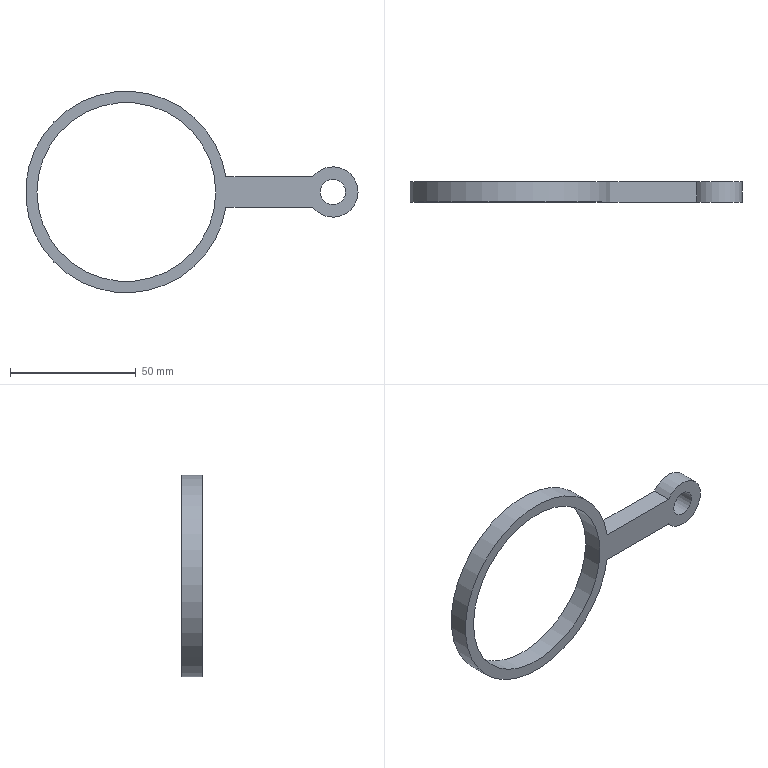Component | NX | ECCENTRIC_ROD | 1 solid | 8 faces | box 132 x 8 x 80 mm | volume 13571 mm3 | cylinder 4 | plane 4 | commonest cylinder face diameters 80 x1 20 x1 71 x1 10 x1
STEP:
#1=CARTESIAN_POINT('',(0.,0.,0.));
#2=DIRECTION('',(0.,0.,1.));
#3=DIRECTION('',(1.,0.,0.));
#4=AXIS2_PLACEMENT_3D('',#1,#2,#3);
#5=CARTESIAN_POINT('',(-111.854,-17.005,113.207));
#6=VERTEX_POINT('',#5);
#7=CARTESIAN_POINT('',(-111.854,-17.005,101.207));
#8=VERTEX_POINT('',#7);
#9=CARTESIAN_POINT('',(-151.401,-17.005,107.207));
#10=DIRECTION('',(0.,-1.,0.));
#11=DIRECTION('',(1.,0.,0.));
#12=AXIS2_PLACEMENT_3D('',#9,#10,#11);
#13=CIRCLE('',#12,40.);
#14=CARTESIAN_POINT('',(-151.401,-25.005,107.207));
#15=DIRECTION('',(0.,1.,0.));
#16=DIRECTION('',(-1.,0.,0.));
#17=AXIS2_PLACEMENT_3D('',#14,#15,#16);
#18=CYLINDRICAL_SURFACE('',#17,40.);
#19=CARTESIAN_POINT('',(3.142,8.));
#20=DIRECTION('',(-1.,0.));
#21=VECTOR('',#20,1.);
#22=LINE('',#19,#21);
#23=(GEOMETRIC_REPRESENTATION_CONTEXT(2)PARAMETRIC_REPRESENTATION_CONTEXT()REPRESENTATION_CONTEXT('',''));
#24=DEFINITIONAL_REPRESENTATION('',(#22),#23);
#25=PCURVE('',#18,#24);
#26=CARTESIAN_POINT('',(-151.401,-17.005,107.207));
#27=DIRECTION('',(0.,-1.,0.));
#28=DIRECTION('',(1.,0.,0.));
#29=AXIS2_PLACEMENT_3D('',#26,#27,#28);
#30=PLANE('',#29);
#31=CARTESIAN_POINT('',(0.,0.));
#32=DIRECTION('',(1.,0.));
#33=AXIS2_PLACEMENT_2D('',#31,#32);
#34=CIRCLE('',#33,40.);
#35=(GEOMETRIC_REPRESENTATION_CONTEXT(2)PARAMETRIC_REPRESENTATION_CONTEXT()REPRESENTATION_CONTEXT('',''));
#36=DEFINITIONAL_REPRESENTATION('',(#34),#35);
#37=PCURVE('',#30,#36);
#38=SURFACE_CURVE('',#13,(#25,#37),.PCURVE_S1.);
#39=EDGE_CURVE('',#6,#8,#38,.T.);
#40=ORIENTED_EDGE('',*,*,#39,.T.);
#41=CARTESIAN_POINT('',(-111.854,-25.005,101.207));
#42=VERTEX_POINT('',#41);
#43=CARTESIAN_POINT('',(-111.854,-25.005,101.207));
#44=DIRECTION('',(0.,1.,0.));
#45=VECTOR('',#44,1.);
#46=LINE('',#43,#45);
#47=CARTESIAN_POINT('',(-2.991,0.));
#48=DIRECTION('',(0.,1.));
#49=VECTOR('',#48,1.);
#50=LINE('',#47,#49);
#51=(GEOMETRIC_REPRESENTATION_CONTEXT(2)PARAMETRIC_REPRESENTATION_CONTEXT()REPRESENTATION_CONTEXT('',''));
#52=DEFINITIONAL_REPRESENTATION('',(#50),#51);
#53=PCURVE('',#18,#52);
#54=CARTESIAN_POINT('',(-111.854,-25.005,101.207));
#55=DIRECTION('',(-0.,0.,1.));
#56=DIRECTION('',(-1.,0.,-0.));
#57=AXIS2_PLACEMENT_3D('',#54,#55,#56);
#58=PLANE('',#57);
#59=CARTESIAN_POINT('',(0.,0.));
#60=DIRECTION('',(0.,-1.));
#61=VECTOR('',#60,1.);
#62=LINE('',#59,#61);
#63=(GEOMETRIC_REPRESENTATION_CONTEXT(2)PARAMETRIC_REPRESENTATION_CONTEXT()REPRESENTATION_CONTEXT('',''));
#64=DEFINITIONAL_REPRESENTATION('',(#62),#63);
#65=PCURVE('',#58,#64);
#66=SURFACE_CURVE('',#46,(#53,#65),.PCURVE_S1.);
#67=EDGE_CURVE('',#42,#8,#66,.T.);
#68=ORIENTED_EDGE('',*,*,#67,.F.);
#69=CARTESIAN_POINT('',(-111.854,-25.005,113.207));
#70=VERTEX_POINT('',#69);
#71=CARTESIAN_POINT('',(-151.401,-25.005,107.207));
#72=DIRECTION('',(0.,-1.,0.));
#73=DIRECTION('',(1.,0.,0.));
#74=AXIS2_PLACEMENT_3D('',#71,#72,#73);
#75=CIRCLE('',#74,40.);
#76=CARTESIAN_POINT('',(3.142,0.));
#77=DIRECTION('',(-1.,0.));
#78=VECTOR('',#77,1.);
#79=LINE('',#76,#78);
#80=(GEOMETRIC_REPRESENTATION_CONTEXT(2)PARAMETRIC_REPRESENTATION_CONTEXT()REPRESENTATION_CONTEXT('',''));
#81=DEFINITIONAL_REPRESENTATION('',(#79),#80);
#82=PCURVE('',#18,#81);
#83=CARTESIAN_POINT('',(-151.401,-25.005,107.207));
#84=DIRECTION('',(0.,-1.,0.));
#85=DIRECTION('',(1.,0.,0.));
#86=AXIS2_PLACEMENT_3D('',#83,#84,#85);
#87=PLANE('',#86);
#88=CARTESIAN_POINT('',(0.,0.));
#89=DIRECTION('',(1.,0.));
#90=AXIS2_PLACEMENT_2D('',#88,#89);
#91=CIRCLE('',#90,40.);
#92=(GEOMETRIC_REPRESENTATION_CONTEXT(2)PARAMETRIC_REPRESENTATION_CONTEXT()REPRESENTATION_CONTEXT('',''));
#93=DEFINITIONAL_REPRESENTATION('',(#91),#92);
#94=PCURVE('',#87,#93);
#95=SURFACE_CURVE('',#75,(#82,#94),.PCURVE_S1.);
#96=EDGE_CURVE('',#70,#42,#95,.T.);
#97=ORIENTED_EDGE('',*,*,#96,.F.);
#98=CARTESIAN_POINT('',(-111.854,-25.005,113.207));
#99=DIRECTION('',(0.,1.,0.));
#100=VECTOR('',#99,1.);
#101=LINE('',#98,#100);
#102=CARTESIAN_POINT('',(2.991,0.));
#103=DIRECTION('',(0.,1.));
#104=VECTOR('',#103,1.);
#105=LINE('',#102,#104);
#106=(GEOMETRIC_REPRESENTATION_CONTEXT(2)PARAMETRIC_REPRESENTATION_CONTEXT()REPRESENTATION_CONTEXT('',''));
#107=DEFINITIONAL_REPRESENTATION('',(#105),#106);
#108=PCURVE('',#18,#107);
#109=CARTESIAN_POINT('',(-77.401,-25.005,113.207));
#110=DIRECTION('',(0.,0.,-1.));
#111=DIRECTION('',(0.,1.,0.));
#112=AXIS2_PLACEMENT_3D('',#109,#110,#111);
#113=PLANE('',#112);
#114=CARTESIAN_POINT('',(0.,-34.453));
#115=DIRECTION('',(1.,0.));
#116=VECTOR('',#115,1.);
#117=LINE('',#114,#116);
#118=(GEOMETRIC_REPRESENTATION_CONTEXT(2)PARAMETRIC_REPRESENTATION_CONTEXT()REPRESENTATION_CONTEXT('',''));
#119=DEFINITIONAL_REPRESENTATION('',(#117),#118);
#120=PCURVE('',#113,#119);
#121=SURFACE_CURVE('',#101,(#108,#120),.PCURVE_S1.);
#122=EDGE_CURVE('',#70,#6,#121,.T.);
#123=ORIENTED_EDGE('',*,*,#122,.T.);
#124=EDGE_LOOP('',(#40,#68,#97,#123));
#125=FACE_BOUND('',#124,.T.);
#126=ADVANCED_FACE('',(#125),#18,.T.);
#127=CARTESIAN_POINT('',(-77.401,-17.005,101.207));
#128=VERTEX_POINT('',#127);
#129=CARTESIAN_POINT('',(-111.854,-17.005,101.207));
#130=DIRECTION('',(1.,0.,0.));
#131=VECTOR('',#130,1.);
#132=LINE('',#129,#131);
#133=CARTESIAN_POINT('',(0.,-8.));
#134=DIRECTION('',(-1.,0.));
#135=VECTOR('',#134,1.);
#136=LINE('',#133,#135);
#137=(GEOMETRIC_REPRESENTATION_CONTEXT(2)PARAMETRIC_REPRESENTATION_CONTEXT()REPRESENTATION_CONTEXT('',''));
#138=DEFINITIONAL_REPRESENTATION('',(#136),#137);
#139=PCURVE('',#58,#138);
#140=CARTESIAN_POINT('',(39.547,-6.));
#141=DIRECTION('',(1.,0.));
#142=VECTOR('',#141,1.);
#143=LINE('',#140,#142);
#144=(GEOMETRIC_REPRESENTATION_CONTEXT(2)PARAMETRIC_REPRESENTATION_CONTEXT()REPRESENTATION_CONTEXT('',''));
#145=DEFINITIONAL_REPRESENTATION('',(#143),#144);
#146=PCURVE('',#30,#145);
#147=SURFACE_CURVE('',#132,(#139,#146),.PCURVE_S1.);
#148=EDGE_CURVE('',#8,#128,#147,.T.);
#149=ORIENTED_EDGE('',*,*,#148,.T.);
#150=CARTESIAN_POINT('',(-77.401,-25.005,101.207));
#151=VERTEX_POINT('',#150);
#152=CARTESIAN_POINT('',(-77.401,-25.005,101.207));
#153=DIRECTION('',(0.,1.,0.));
#154=VECTOR('',#153,1.);
#155=LINE('',#152,#154);
#156=CARTESIAN_POINT('',(-34.453,0.));
#157=DIRECTION('',(0.,-1.));
#158=VECTOR('',#157,1.);
#159=LINE('',#156,#158);
#160=(GEOMETRIC_REPRESENTATION_CONTEXT(2)PARAMETRIC_REPRESENTATION_CONTEXT()REPRESENTATION_CONTEXT('',''));
#161=DEFINITIONAL_REPRESENTATION('',(#159),#160);
#162=PCURVE('',#58,#161);
#163=CARTESIAN_POINT('',(-69.401,-25.005,107.207));
#164=DIRECTION('',(0.,1.,0.));
#165=DIRECTION('',(-1.,0.,0.));
#166=AXIS2_PLACEMENT_3D('',#163,#164,#165);
#167=CYLINDRICAL_SURFACE('',#166,10.);
#168=CARTESIAN_POINT('',(5.64,0.));
#169=DIRECTION('',(0.,1.));
#170=VECTOR('',#169,1.);
#171=LINE('',#168,#170);
#172=(GEOMETRIC_REPRESENTATION_CONTEXT(2)PARAMETRIC_REPRESENTATION_CONTEXT()REPRESENTATION_CONTEXT('',''));
#173=DEFINITIONAL_REPRESENTATION('',(#171),#172);
#174=PCURVE('',#167,#173);
#175=SURFACE_CURVE('',#155,(#162,#174),.PCURVE_S1.);
#176=EDGE_CURVE('',#151,#128,#175,.T.);
#177=ORIENTED_EDGE('',*,*,#176,.F.);
#178=CARTESIAN_POINT('',(-111.854,-25.005,101.207));
#179=DIRECTION('',(1.,0.,0.));
#180=VECTOR('',#179,1.);
#181=LINE('',#178,#180);
#182=CARTESIAN_POINT('',(0.,0.));
#183=DIRECTION('',(-1.,0.));
#184=VECTOR('',#183,1.);
#185=LINE('',#182,#184);
#186=(GEOMETRIC_REPRESENTATION_CONTEXT(2)PARAMETRIC_REPRESENTATION_CONTEXT()REPRESENTATION_CONTEXT('',''));
#187=DEFINITIONAL_REPRESENTATION('',(#185),#186);
#188=PCURVE('',#58,#187);
#189=CARTESIAN_POINT('',(39.547,-6.));
#190=DIRECTION('',(1.,0.));
#191=VECTOR('',#190,1.);
#192=LINE('',#189,#191);
#193=(GEOMETRIC_REPRESENTATION_CONTEXT(2)PARAMETRIC_REPRESENTATION_CONTEXT()REPRESENTATION_CONTEXT('',''));
#194=DEFINITIONAL_REPRESENTATION('',(#192),#193);
#195=PCURVE('',#87,#194);
#196=SURFACE_CURVE('',#181,(#188,#195),.PCURVE_S1.);
#197=EDGE_CURVE('',#42,#151,#196,.T.);
#198=ORIENTED_EDGE('',*,*,#197,.F.);
#199=ORIENTED_EDGE('',*,*,#67,.T.);
#200=EDGE_LOOP('',(#149,#177,#198,#199));
#201=FACE_BOUND('',#200,.T.);
#202=ADVANCED_FACE('',(#201),#58,.F.);
#203=CARTESIAN_POINT('',(-77.401,-17.005,113.207));
#204=VERTEX_POINT('',#203);
#205=CARTESIAN_POINT('',(-69.401,-17.005,107.207));
#206=DIRECTION('',(0.,-1.,0.));
#207=DIRECTION('',(1.,0.,0.));
#208=AXIS2_PLACEMENT_3D('',#205,#206,#207);
#209=CIRCLE('',#208,10.);
#210=CARTESIAN_POINT('',(9.425,8.));
#211=DIRECTION('',(-1.,0.));
#212=VECTOR('',#211,1.);
#213=LINE('',#210,#212);
#214=(GEOMETRIC_REPRESENTATION_CONTEXT(2)PARAMETRIC_REPRESENTATION_CONTEXT()REPRESENTATION_CONTEXT('',''));
#215=DEFINITIONAL_REPRESENTATION('',(#213),#214);
#216=PCURVE('',#167,#215);
#217=CARTESIAN_POINT('',(82.,0.));
#218=DIRECTION('',(1.,0.));
#219=AXIS2_PLACEMENT_2D('',#217,#218);
#220=CIRCLE('',#219,10.);
#221=(GEOMETRIC_REPRESENTATION_CONTEXT(2)PARAMETRIC_REPRESENTATION_CONTEXT()REPRESENTATION_CONTEXT('',''));
#222=DEFINITIONAL_REPRESENTATION('',(#220),#221);
#223=PCURVE('',#30,#222);
#224=SURFACE_CURVE('',#209,(#216,#223),.PCURVE_S1.);
#225=EDGE_CURVE('',#128,#204,#224,.T.);
#226=ORIENTED_EDGE('',*,*,#225,.T.);
#227=CARTESIAN_POINT('',(-77.401,-25.005,113.207));
#228=VERTEX_POINT('',#227);
#229=CARTESIAN_POINT('',(-77.401,-25.005,113.207));
#230=DIRECTION('',(0.,1.,0.));
#231=VECTOR('',#230,1.);
#232=LINE('',#229,#231);
#233=CARTESIAN_POINT('',(0.6435,0.));
#234=DIRECTION('',(0.,1.));
#235=VECTOR('',#234,1.);
#236=LINE('',#233,#235);
#237=(GEOMETRIC_REPRESENTATION_CONTEXT(2)PARAMETRIC_REPRESENTATION_CONTEXT()REPRESENTATION_CONTEXT('',''));
#238=DEFINITIONAL_REPRESENTATION('',(#236),#237);
#239=PCURVE('',#167,#238);
#240=CARTESIAN_POINT('',(0.,0.));
#241=DIRECTION('',(1.,0.));
#242=VECTOR('',#241,1.);
#243=LINE('',#240,#242);
#244=(GEOMETRIC_REPRESENTATION_CONTEXT(2)PARAMETRIC_REPRESENTATION_CONTEXT()REPRESENTATION_CONTEXT('',''));
#245=DEFINITIONAL_REPRESENTATION('',(#243),#244);
#246=PCURVE('',#113,#245);
#247=SURFACE_CURVE('',#232,(#239,#246),.PCURVE_S1.);
#248=EDGE_CURVE('',#228,#204,#247,.T.);
#249=ORIENTED_EDGE('',*,*,#248,.F.);
#250=CARTESIAN_POINT('',(-69.401,-25.005,107.207));
#251=DIRECTION('',(0.,-1.,0.));
#252=DIRECTION('',(1.,0.,0.));
#253=AXIS2_PLACEMENT_3D('',#250,#251,#252);
#254=CIRCLE('',#253,10.);
#255=CARTESIAN_POINT('',(9.425,0.));
#256=DIRECTION('',(-1.,0.));
#257=VECTOR('',#256,1.);
#258=LINE('',#255,#257);
#259=(GEOMETRIC_REPRESENTATION_CONTEXT(2)PARAMETRIC_REPRESENTATION_CONTEXT()REPRESENTATION_CONTEXT('',''));
#260=DEFINITIONAL_REPRESENTATION('',(#258),#259);
#261=PCURVE('',#167,#260);
#262=CARTESIAN_POINT('',(82.,0.));
#263=DIRECTION('',(1.,0.));
#264=AXIS2_PLACEMENT_2D('',#262,#263);
#265=CIRCLE('',#264,10.);
#266=(GEOMETRIC_REPRESENTATION_CONTEXT(2)PARAMETRIC_REPRESENTATION_CONTEXT()REPRESENTATION_CONTEXT('',''));
#267=DEFINITIONAL_REPRESENTATION('',(#265),#266);
#268=PCURVE('',#87,#267);
#269=SURFACE_CURVE('',#254,(#261,#268),.PCURVE_S1.);
#270=EDGE_CURVE('',#151,#228,#269,.T.);
#271=ORIENTED_EDGE('',*,*,#270,.F.);
#272=ORIENTED_EDGE('',*,*,#176,.T.);
#273=EDGE_LOOP('',(#226,#249,#271,#272));
#274=FACE_BOUND('',#273,.T.);
#275=ADVANCED_FACE('',(#274),#167,.T.);
#276=CARTESIAN_POINT('',(-115.901,-25.005,107.207));
#277=VERTEX_POINT('',#276);
#278=CARTESIAN_POINT('',(-151.401,-25.005,107.207));
#279=DIRECTION('',(0.,-1.,0.));
#280=DIRECTION('',(1.,0.,0.));
#281=AXIS2_PLACEMENT_3D('',#278,#279,#280);
#282=CIRCLE('',#281,35.5);
#283=CARTESIAN_POINT('',(-151.401,-25.005,107.207));
#284=DIRECTION('',(0.,1.,0.));
#285=DIRECTION('',(-1.,0.,0.));
#286=AXIS2_PLACEMENT_3D('',#283,#284,#285);
#287=CYLINDRICAL_SURFACE('',#286,35.5);
#288=CARTESIAN_POINT('',(9.425,0.));
#289=DIRECTION('',(-1.,0.));
#290=VECTOR('',#289,1.);
#291=LINE('',#288,#290);
#292=(GEOMETRIC_REPRESENTATION_CONTEXT(2)PARAMETRIC_REPRESENTATION_CONTEXT()REPRESENTATION_CONTEXT('',''));
#293=DEFINITIONAL_REPRESENTATION('',(#291),#292);
#294=PCURVE('',#287,#293);
#295=CARTESIAN_POINT('',(0.,0.));
#296=DIRECTION('',(1.,0.));
#297=AXIS2_PLACEMENT_2D('',#295,#296);
#298=CIRCLE('',#297,35.5);
#299=(GEOMETRIC_REPRESENTATION_CONTEXT(2)PARAMETRIC_REPRESENTATION_CONTEXT()REPRESENTATION_CONTEXT('',''));
#300=DEFINITIONAL_REPRESENTATION('',(#298),#299);
#301=PCURVE('',#87,#300);
#302=SURFACE_CURVE('',#282,(#294,#301),.PCURVE_S1.);
#303=EDGE_CURVE('',#277,#277,#302,.T.);
#304=ORIENTED_EDGE('',*,*,#303,.F.);
#305=CARTESIAN_POINT('',(-115.901,-17.005,107.207));
#306=VERTEX_POINT('',#305);
#307=CARTESIAN_POINT('',(-115.901,-25.005,107.207));
#308=CARTESIAN_POINT('',(-115.901,-17.005,107.207));
#309=B_SPLINE_CURVE_WITH_KNOTS('',1,(#307,#308),.UNSPECIFIED.,.F.,.F.,(2,2),(0.,8.),.PIECEWISE_BEZIER_KNOTS.);
#310=CARTESIAN_POINT('',(9.425,0.));
#311=DIRECTION('',(0.,1.));
#312=VECTOR('',#311,1.);
#313=LINE('',#310,#312);
#314=(GEOMETRIC_REPRESENTATION_CONTEXT(2)PARAMETRIC_REPRESENTATION_CONTEXT()REPRESENTATION_CONTEXT('',''));
#315=DEFINITIONAL_REPRESENTATION('',(#313),#314);
#316=PCURVE('',#287,#315);
#317=CARTESIAN_POINT('',(3.142,0.));
#318=DIRECTION('',(0.,1.));
#319=VECTOR('',#318,1.);
#320=LINE('',#317,#319);
#321=(GEOMETRIC_REPRESENTATION_CONTEXT(2)PARAMETRIC_REPRESENTATION_CONTEXT()REPRESENTATION_CONTEXT('',''));
#322=DEFINITIONAL_REPRESENTATION('',(#320),#321);
#323=PCURVE('',#287,#322);
#324=SEAM_CURVE('',#309,(#316,#323),.PCURVE_S1.);
#325=EDGE_CURVE('',#277,#306,#324,.T.);
#326=ORIENTED_EDGE('',*,*,#325,.T.);
#327=CARTESIAN_POINT('',(-151.401,-17.005,107.207));
#328=DIRECTION('',(0.,-1.,0.));
#329=DIRECTION('',(1.,0.,0.));
#330=AXIS2_PLACEMENT_3D('',#327,#328,#329);
#331=CIRCLE('',#330,35.5);
#332=CARTESIAN_POINT('',(9.425,8.));
#333=DIRECTION('',(-1.,0.));
#334=VECTOR('',#333,1.);
#335=LINE('',#332,#334);
#336=(GEOMETRIC_REPRESENTATION_CONTEXT(2)PARAMETRIC_REPRESENTATION_CONTEXT()REPRESENTATION_CONTEXT('',''));
#337=DEFINITIONAL_REPRESENTATION('',(#335),#336);
#338=PCURVE('',#287,#337);
#339=CARTESIAN_POINT('',(0.,0.));
#340=DIRECTION('',(1.,0.));
#341=AXIS2_PLACEMENT_2D('',#339,#340);
#342=CIRCLE('',#341,35.5);
#343=(GEOMETRIC_REPRESENTATION_CONTEXT(2)PARAMETRIC_REPRESENTATION_CONTEXT()REPRESENTATION_CONTEXT('',''));
#344=DEFINITIONAL_REPRESENTATION('',(#342),#343);
#345=PCURVE('',#30,#344);
#346=SURFACE_CURVE('',#331,(#338,#345),.PCURVE_S1.);
#347=EDGE_CURVE('',#306,#306,#346,.T.);
#348=ORIENTED_EDGE('',*,*,#347,.T.);
#349=ORIENTED_EDGE('',*,*,#325,.F.);
#350=EDGE_LOOP('',(#304,#326,#348,#349));
#351=FACE_BOUND('',#350,.F.);
#352=ADVANCED_FACE('',(#351),#287,.F.);
#353=CARTESIAN_POINT('',(-77.401,-17.005,113.207));
#354=DIRECTION('',(-1.,0.,0.));
#355=VECTOR('',#354,1.);
#356=LINE('',#353,#355);
#357=CARTESIAN_POINT('',(8.,0.));
#358=DIRECTION('',(0.,-1.));
#359=VECTOR('',#358,1.);
#360=LINE('',#357,#359);
#361=(GEOMETRIC_REPRESENTATION_CONTEXT(2)PARAMETRIC_REPRESENTATION_CONTEXT()REPRESENTATION_CONTEXT('',''));
#362=DEFINITIONAL_REPRESENTATION('',(#360),#361);
#363=PCURVE('',#113,#362);
#364=CARTESIAN_POINT('',(74.,6.));
#365=DIRECTION('',(-1.,0.));
#366=VECTOR('',#365,1.);
#367=LINE('',#364,#366);
#368=(GEOMETRIC_REPRESENTATION_CONTEXT(2)PARAMETRIC_REPRESENTATION_CONTEXT()REPRESENTATION_CONTEXT('',''));
#369=DEFINITIONAL_REPRESENTATION('',(#367),#368);
#370=PCURVE('',#30,#369);
#371=SURFACE_CURVE('',#356,(#363,#370),.PCURVE_S1.);
#372=EDGE_CURVE('',#204,#6,#371,.T.);
#373=ORIENTED_EDGE('',*,*,#372,.T.);
#374=ORIENTED_EDGE('',*,*,#122,.F.);
#375=CARTESIAN_POINT('',(-77.401,-25.005,113.207));
#376=DIRECTION('',(-1.,0.,0.));
#377=VECTOR('',#376,1.);
#378=LINE('',#375,#377);
#379=CARTESIAN_POINT('',(0.,0.));
#380=DIRECTION('',(0.,-1.));
#381=VECTOR('',#380,1.);
#382=LINE('',#379,#381);
#383=(GEOMETRIC_REPRESENTATION_CONTEXT(2)PARAMETRIC_REPRESENTATION_CONTEXT()REPRESENTATION_CONTEXT('',''));
#384=DEFINITIONAL_REPRESENTATION('',(#382),#383);
#385=PCURVE('',#113,#384);
#386=CARTESIAN_POINT('',(74.,6.));
#387=DIRECTION('',(-1.,0.));
#388=VECTOR('',#387,1.);
#389=LINE('',#386,#388);
#390=(GEOMETRIC_REPRESENTATION_CONTEXT(2)PARAMETRIC_REPRESENTATION_CONTEXT()REPRESENTATION_CONTEXT('',''));
#391=DEFINITIONAL_REPRESENTATION('',(#389),#390);
#392=PCURVE('',#87,#391);
#393=SURFACE_CURVE('',#378,(#385,#392),.PCURVE_S1.);
#394=EDGE_CURVE('',#228,#70,#393,.T.);
#395=ORIENTED_EDGE('',*,*,#394,.F.);
#396=ORIENTED_EDGE('',*,*,#248,.T.);
#397=EDGE_LOOP('',(#373,#374,#395,#396));
#398=FACE_BOUND('',#397,.T.);
#399=ADVANCED_FACE('',(#398),#113,.F.);
#400=CARTESIAN_POINT('',(-64.401,-25.005,107.207));
#401=VERTEX_POINT('',#400);
#402=CARTESIAN_POINT('',(-69.401,-25.005,107.207));
#403=DIRECTION('',(0.,-1.,0.));
#404=DIRECTION('',(1.,0.,0.));
#405=AXIS2_PLACEMENT_3D('',#402,#403,#404);
#406=CIRCLE('',#405,5.);
#407=CARTESIAN_POINT('',(-69.401,-25.005,107.207));
#408=DIRECTION('',(0.,1.,0.));
#409=DIRECTION('',(-1.,0.,0.));
#410=AXIS2_PLACEMENT_3D('',#407,#408,#409);
#411=CYLINDRICAL_SURFACE('',#410,5.);
#412=CARTESIAN_POINT('',(9.425,0.));
#413=DIRECTION('',(-1.,0.));
#414=VECTOR('',#413,1.);
#415=LINE('',#412,#414);
#416=(GEOMETRIC_REPRESENTATION_CONTEXT(2)PARAMETRIC_REPRESENTATION_CONTEXT()REPRESENTATION_CONTEXT('',''));
#417=DEFINITIONAL_REPRESENTATION('',(#415),#416);
#418=PCURVE('',#411,#417);
#419=CARTESIAN_POINT('',(82.,0.));
#420=DIRECTION('',(1.,0.));
#421=AXIS2_PLACEMENT_2D('',#419,#420);
#422=CIRCLE('',#421,5.);
#423=(GEOMETRIC_REPRESENTATION_CONTEXT(2)PARAMETRIC_REPRESENTATION_CONTEXT()REPRESENTATION_CONTEXT('',''));
#424=DEFINITIONAL_REPRESENTATION('',(#422),#423);
#425=PCURVE('',#87,#424);
#426=SURFACE_CURVE('',#406,(#418,#425),.PCURVE_S1.);
#427=EDGE_CURVE('',#401,#401,#426,.T.);
#428=ORIENTED_EDGE('',*,*,#427,.F.);
#429=CARTESIAN_POINT('',(-64.401,-17.005,107.207));
#430=VERTEX_POINT('',#429);
#431=CARTESIAN_POINT('',(-64.401,-25.005,107.207));
#432=CARTESIAN_POINT('',(-64.401,-17.005,107.207));
#433=B_SPLINE_CURVE_WITH_KNOTS('',1,(#431,#432),.UNSPECIFIED.,.F.,.F.,(2,2),(0.,8.),.PIECEWISE_BEZIER_KNOTS.);
#434=CARTESIAN_POINT('',(9.425,0.));
#435=DIRECTION('',(0.,1.));
#436=VECTOR('',#435,1.);
#437=LINE('',#434,#436);
#438=(GEOMETRIC_REPRESENTATION_CONTEXT(2)PARAMETRIC_REPRESENTATION_CONTEXT()REPRESENTATION_CONTEXT('',''));
#439=DEFINITIONAL_REPRESENTATION('',(#437),#438);
#440=PCURVE('',#411,#439);
#441=CARTESIAN_POINT('',(3.142,0.));
#442=DIRECTION('',(0.,1.));
#443=VECTOR('',#442,1.);
#444=LINE('',#441,#443);
#445=(GEOMETRIC_REPRESENTATION_CONTEXT(2)PARAMETRIC_REPRESENTATION_CONTEXT()REPRESENTATION_CONTEXT('',''));
#446=DEFINITIONAL_REPRESENTATION('',(#444),#445);
#447=PCURVE('',#411,#446);
#448=SEAM_CURVE('',#433,(#440,#447),.PCURVE_S1.);
#449=EDGE_CURVE('',#401,#430,#448,.T.);
#450=ORIENTED_EDGE('',*,*,#449,.T.);
#451=CARTESIAN_POINT('',(-69.401,-17.005,107.207));
#452=DIRECTION('',(0.,-1.,0.));
#453=DIRECTION('',(1.,0.,0.));
#454=AXIS2_PLACEMENT_3D('',#451,#452,#453);
#455=CIRCLE('',#454,5.);
#456=CARTESIAN_POINT('',(9.425,8.));
#457=DIRECTION('',(-1.,0.));
#458=VECTOR('',#457,1.);
#459=LINE('',#456,#458);
#460=(GEOMETRIC_REPRESENTATION_CONTEXT(2)PARAMETRIC_REPRESENTATION_CONTEXT()REPRESENTATION_CONTEXT('',''));
#461=DEFINITIONAL_REPRESENTATION('',(#459),#460);
#462=PCURVE('',#411,#461);
#463=CARTESIAN_POINT('',(82.,0.));
#464=DIRECTION('',(1.,0.));
#465=AXIS2_PLACEMENT_2D('',#463,#464);
#466=CIRCLE('',#465,5.);
#467=(GEOMETRIC_REPRESENTATION_CONTEXT(2)PARAMETRIC_REPRESENTATION_CONTEXT()REPRESENTATION_CONTEXT('',''));
#468=DEFINITIONAL_REPRESENTATION('',(#466),#467);
#469=PCURVE('',#30,#468);
#470=SURFACE_CURVE('',#455,(#462,#469),.PCURVE_S1.);
#471=EDGE_CURVE('',#430,#430,#470,.T.);
#472=ORIENTED_EDGE('',*,*,#471,.T.);
#473=ORIENTED_EDGE('',*,*,#449,.F.);
#474=EDGE_LOOP('',(#428,#450,#472,#473));
#475=FACE_BOUND('',#474,.F.);
#476=ADVANCED_FACE('',(#475),#411,.F.);
#477=ORIENTED_EDGE('',*,*,#96,.T.);
#478=ORIENTED_EDGE('',*,*,#197,.T.);
#479=ORIENTED_EDGE('',*,*,#270,.T.);
#480=ORIENTED_EDGE('',*,*,#394,.T.);
#481=EDGE_LOOP('',(#477,#478,#479,#480));
#482=FACE_BOUND('',#481,.T.);
#483=ORIENTED_EDGE('',*,*,#303,.F.);
#484=EDGE_LOOP('',(#483));
#485=FACE_BOUND('',#484,.T.);
#486=ORIENTED_EDGE('',*,*,#427,.F.);
#487=EDGE_LOOP('',(#486));
#488=FACE_BOUND('',#487,.T.);
#489=ADVANCED_FACE('',(#482,#485,#488),#87,.T.);
#490=ORIENTED_EDGE('',*,*,#39,.F.);
#491=ORIENTED_EDGE('',*,*,#372,.F.);
#492=ORIENTED_EDGE('',*,*,#225,.F.);
#493=ORIENTED_EDGE('',*,*,#148,.F.);
#494=EDGE_LOOP('',(#490,#491,#492,#493));
#495=FACE_BOUND('',#494,.T.);
#496=ORIENTED_EDGE('',*,*,#347,.T.);
#497=EDGE_LOOP('',(#496));
#498=FACE_BOUND('',#497,.T.);
#499=ORIENTED_EDGE('',*,*,#471,.T.);
#500=EDGE_LOOP('',(#499));
#501=FACE_BOUND('',#500,.T.);
#502=ADVANCED_FACE('',(#495,#498,#501),#30,.F.);
#503=CLOSED_SHELL('',(#126,#202,#275,#352,#399,#476,#489,#502));
#504=MANIFOLD_SOLID_BREP('',#503);
#505=(LENGTH_UNIT()NAMED_UNIT(*)SI_UNIT(.MILLI.,.METRE.));
#506=UNCERTAINTY_MEASURE_WITH_UNIT(LENGTH_MEASURE(0.000002),#505,'','');
#507=(NAMED_UNIT(*)PLANE_ANGLE_UNIT()SI_UNIT($,.RADIAN.));
#508=(NAMED_UNIT(*)SI_UNIT($,.STERADIAN.)SOLID_ANGLE_UNIT());
#509=(GEOMETRIC_REPRESENTATION_CONTEXT(3)GLOBAL_UNCERTAINTY_ASSIGNED_CONTEXT((#506))GLOBAL_UNIT_ASSIGNED_CONTEXT((#505,#507,#508))REPRESENTATION_CONTEXT('',''));
#510=ADVANCED_BREP_SHAPE_REPRESENTATION('',(#4,#504),#509);